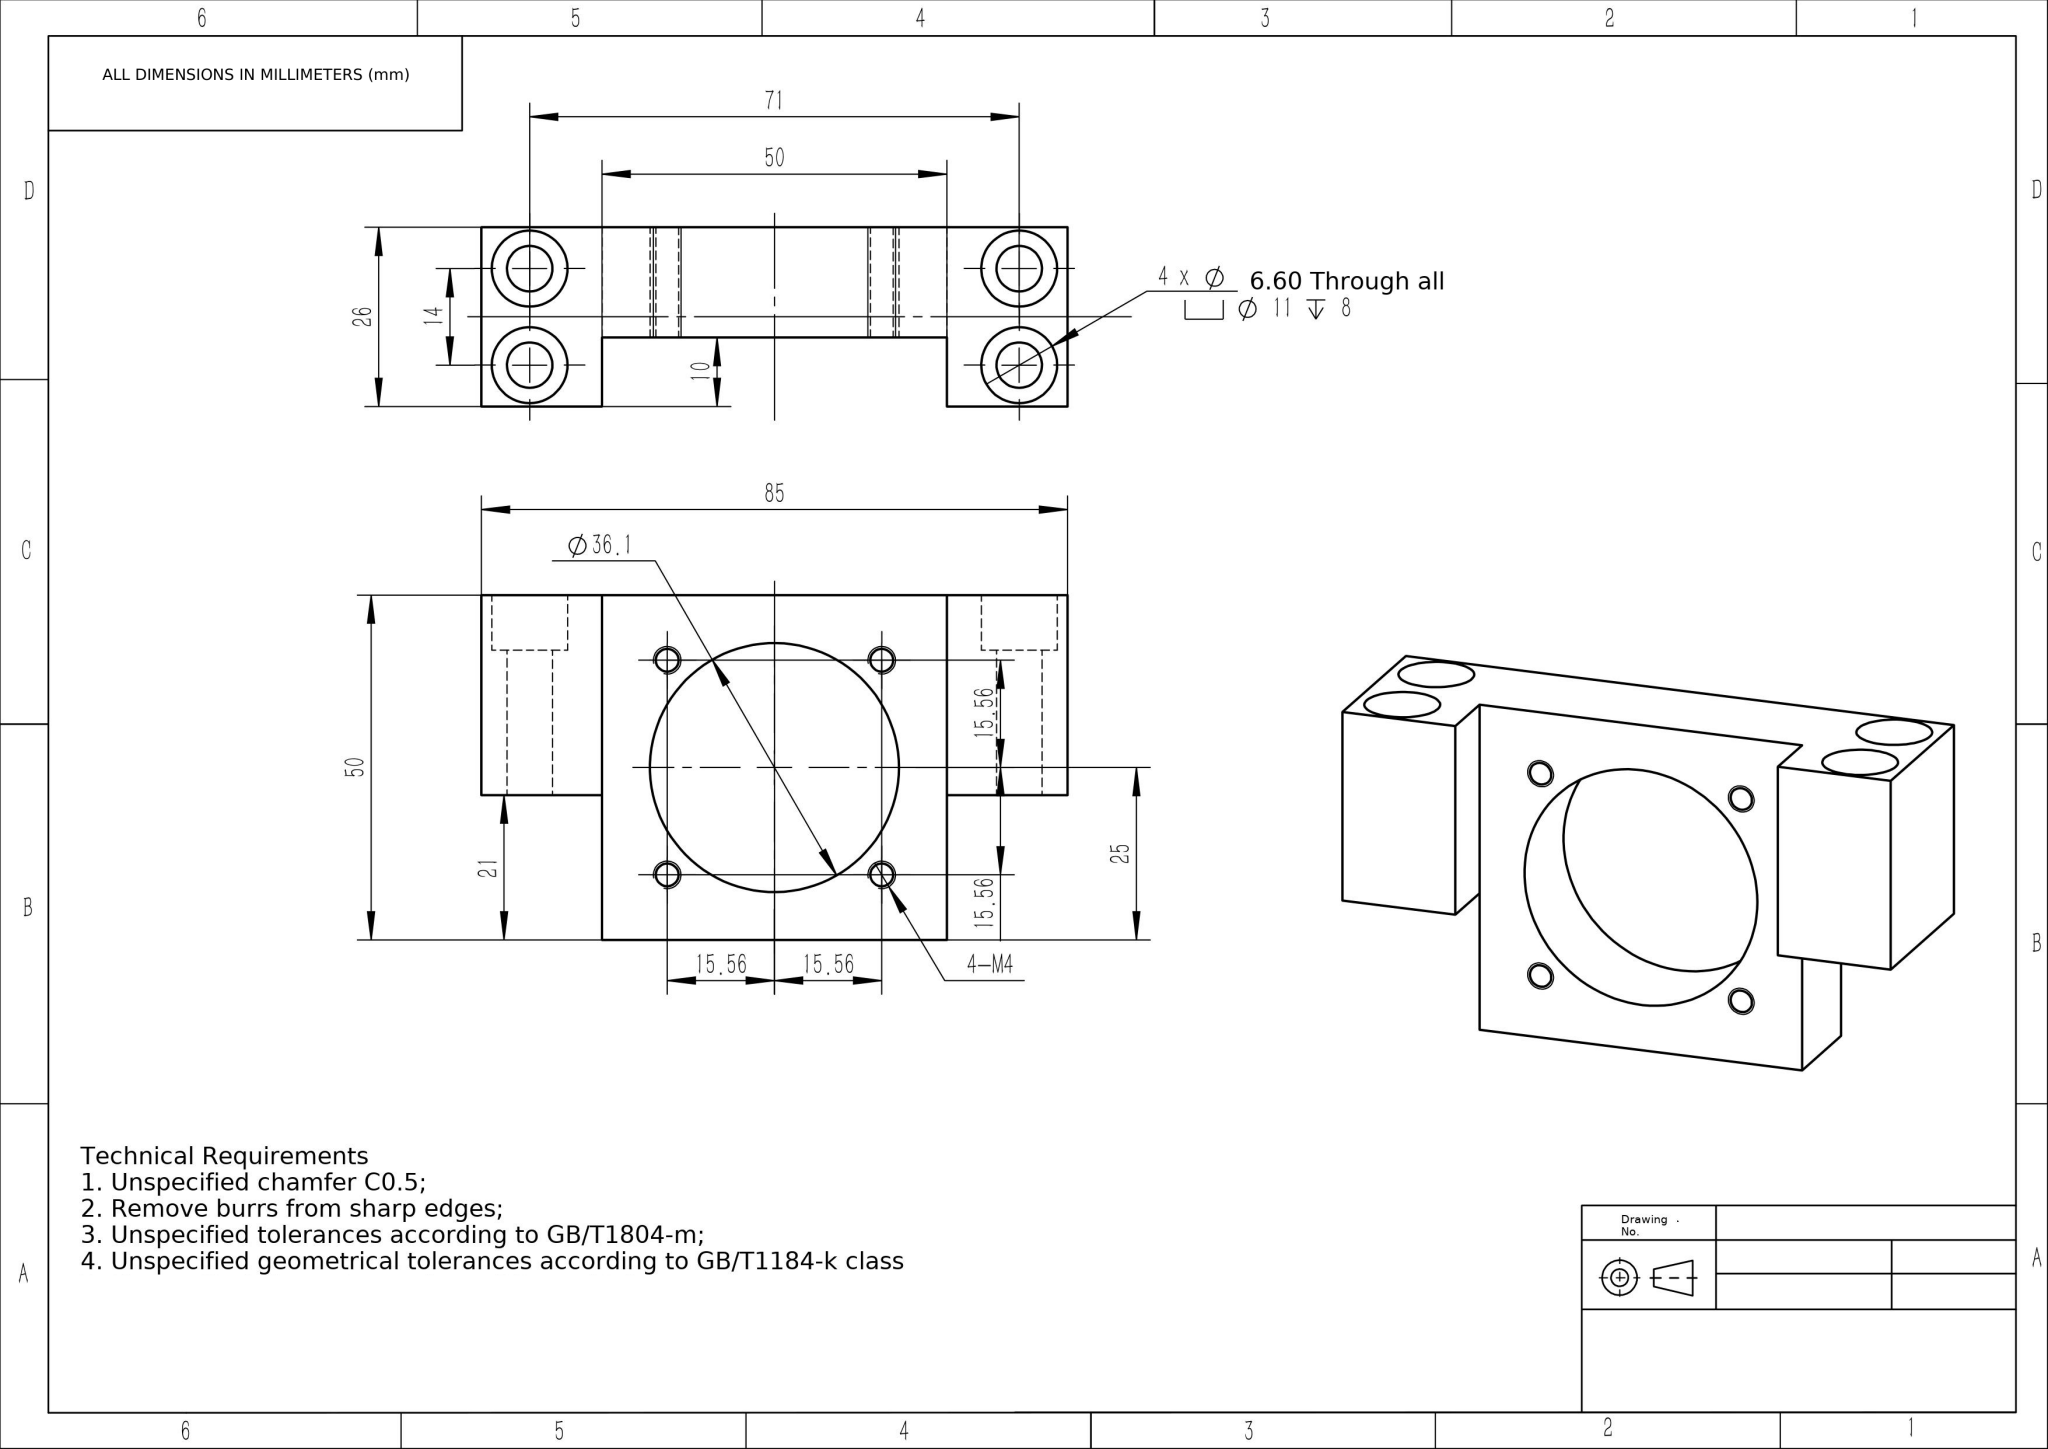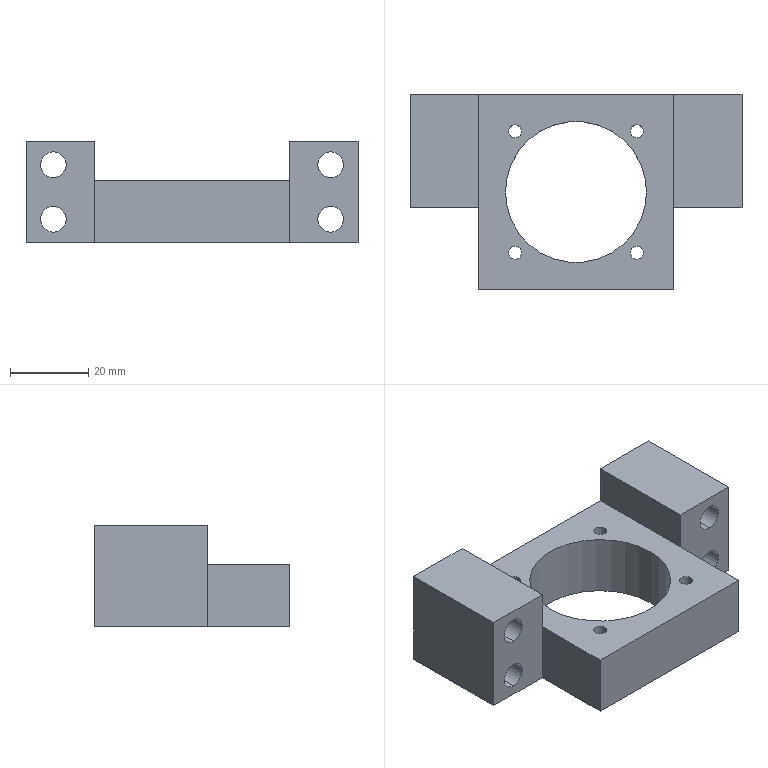Part | NX | mm | 1 solid | 44 faces | box 85 x 50 x 26 mm | volume 43551 mm3 | cylinder 26 | plane 18 | commonest cylinder face diameters 3.3 x8 11 x8 6.6 x8 36.1 x2